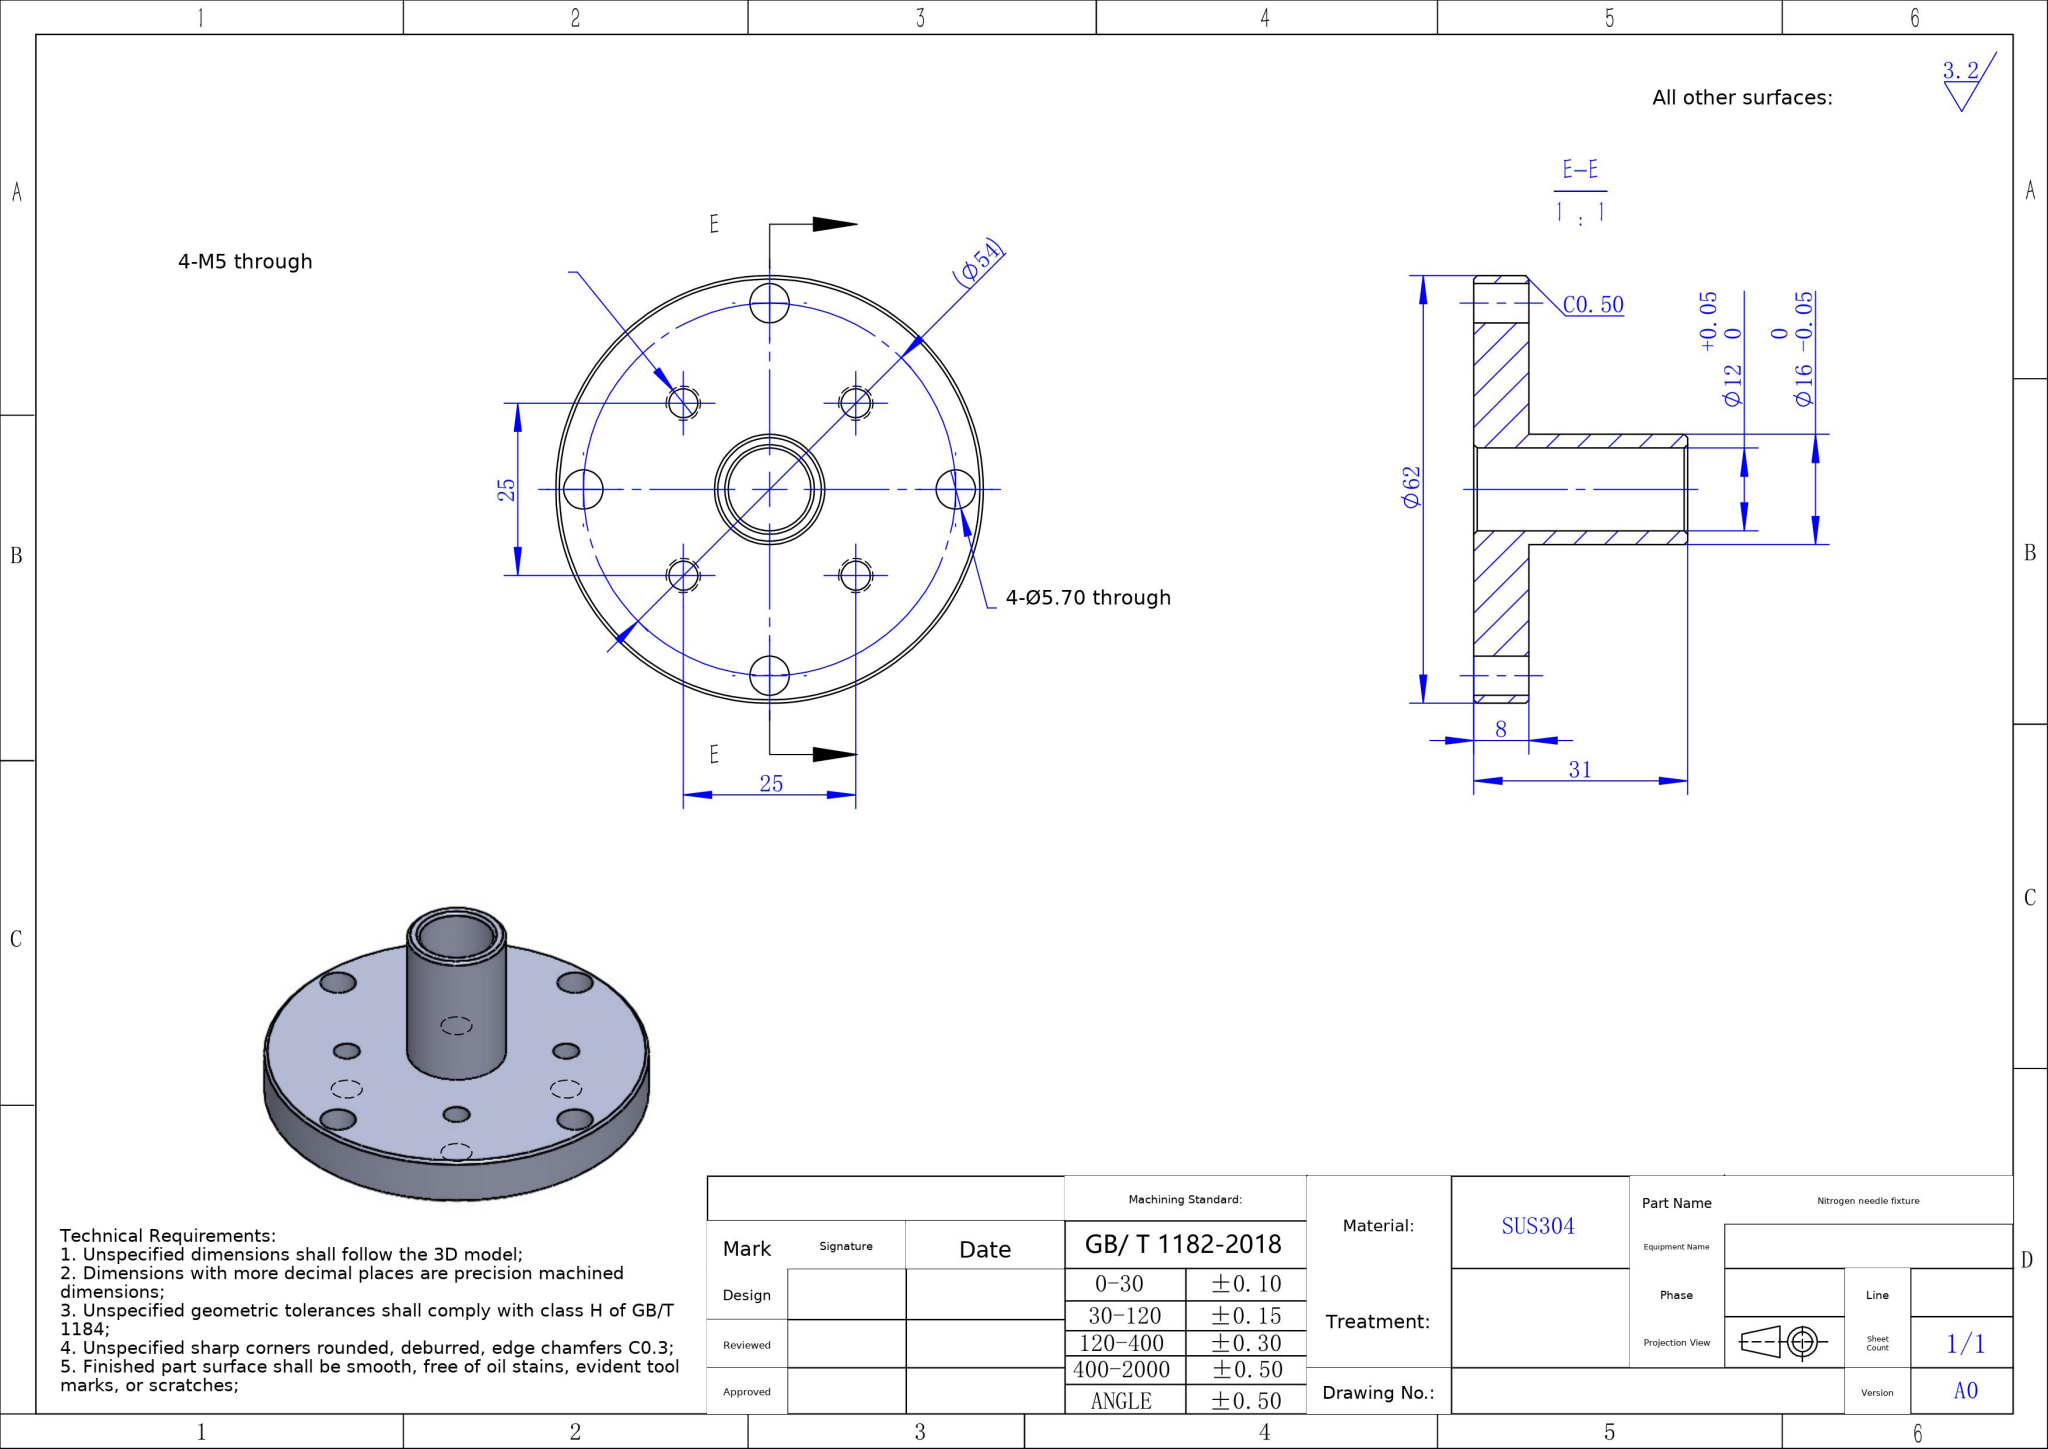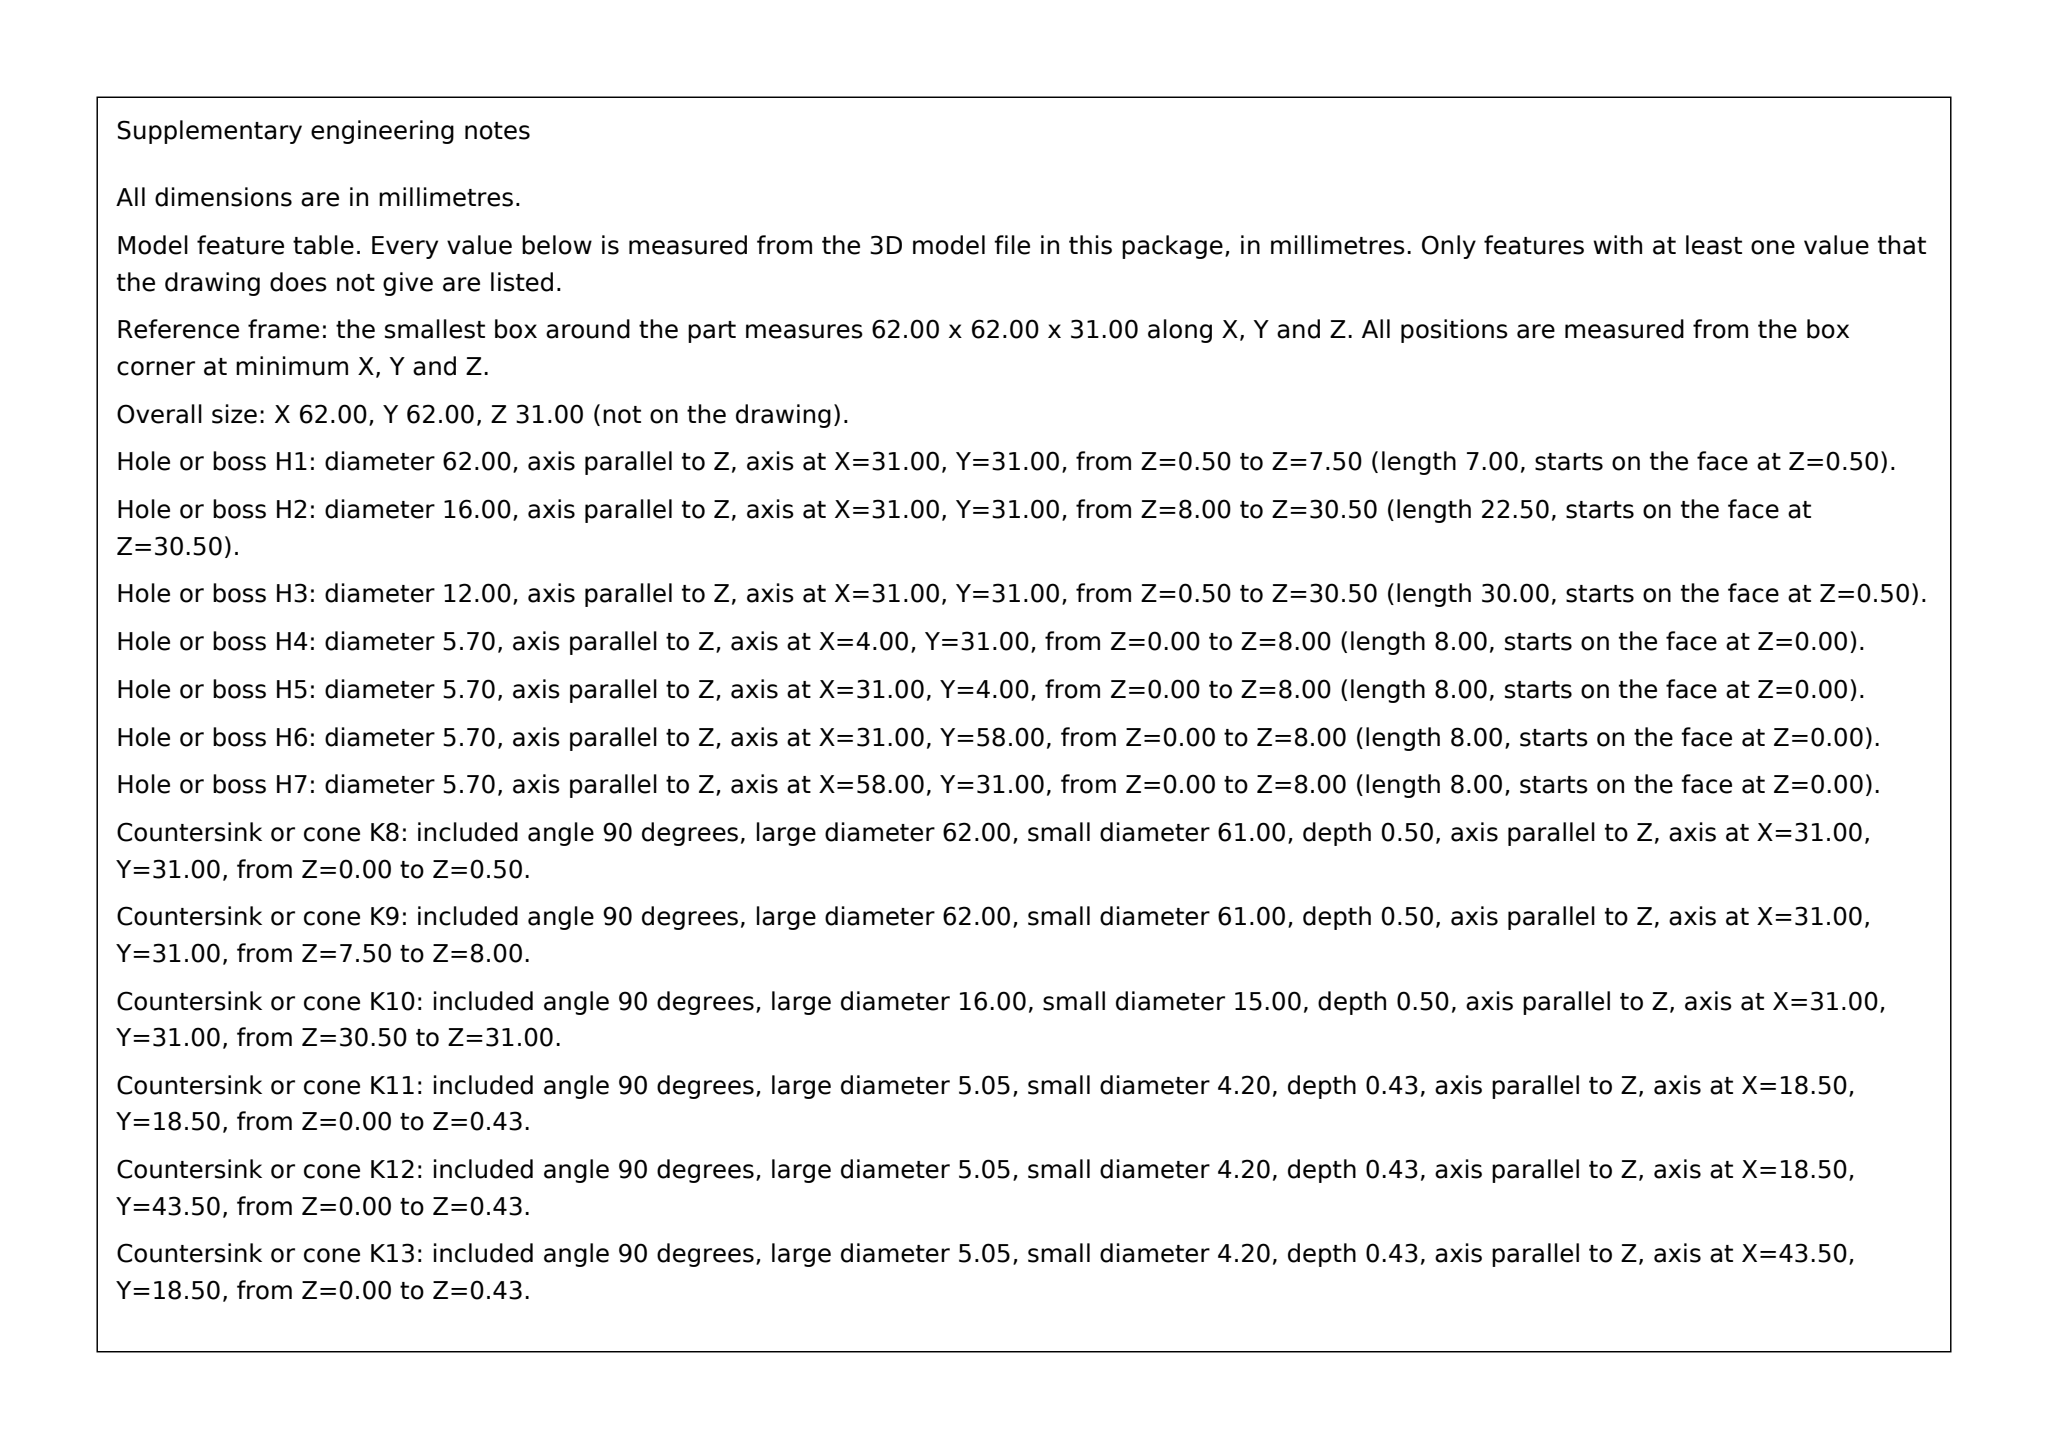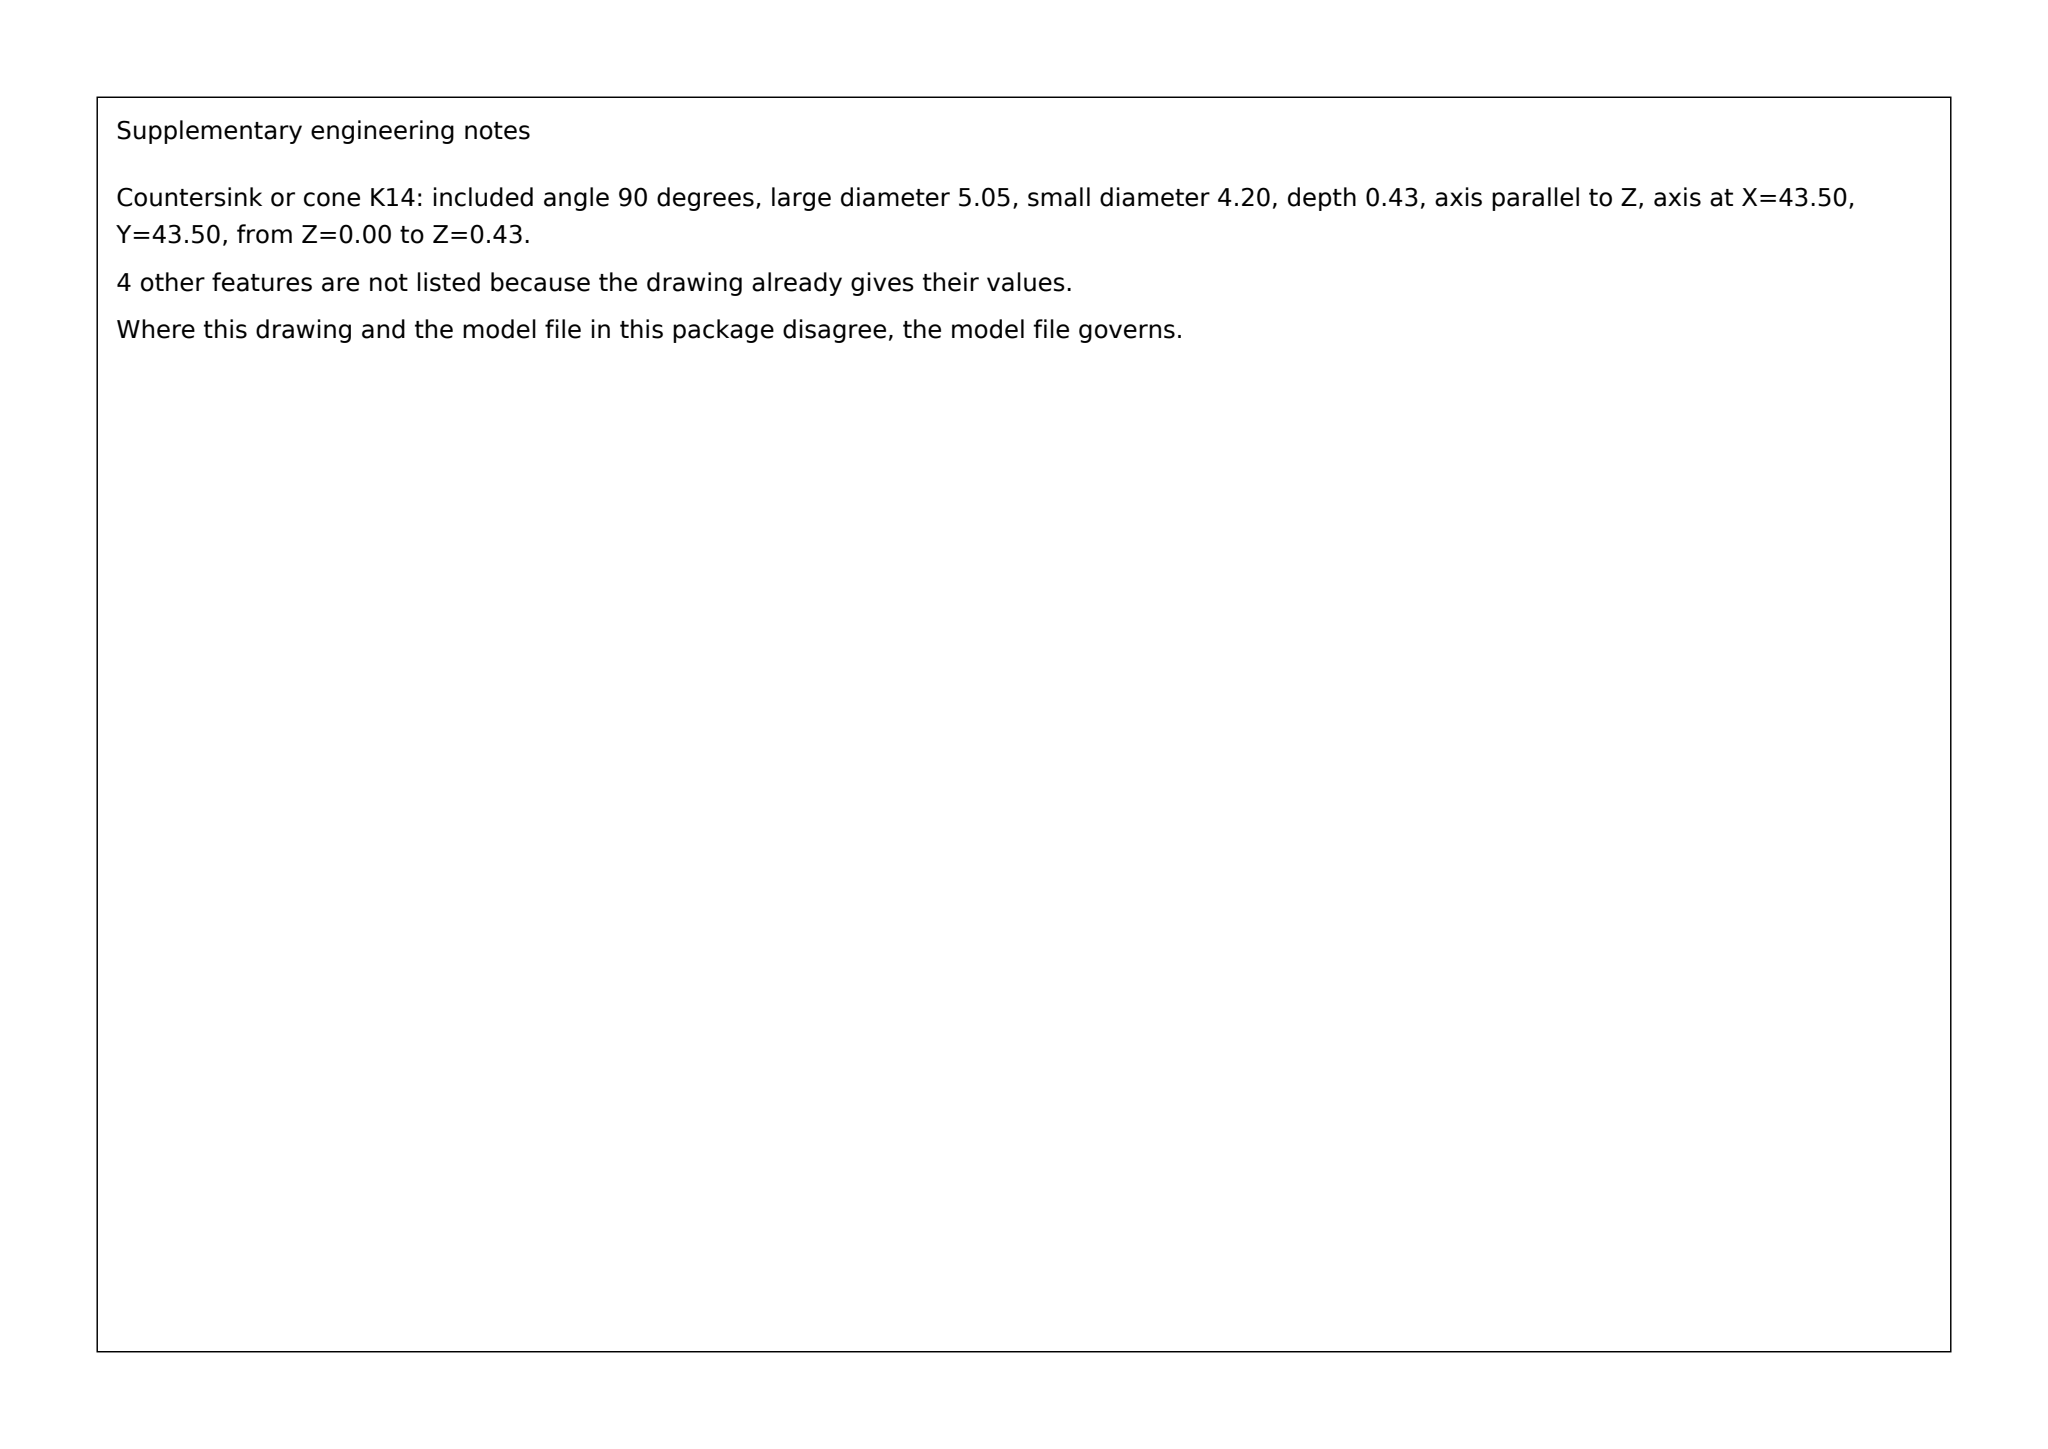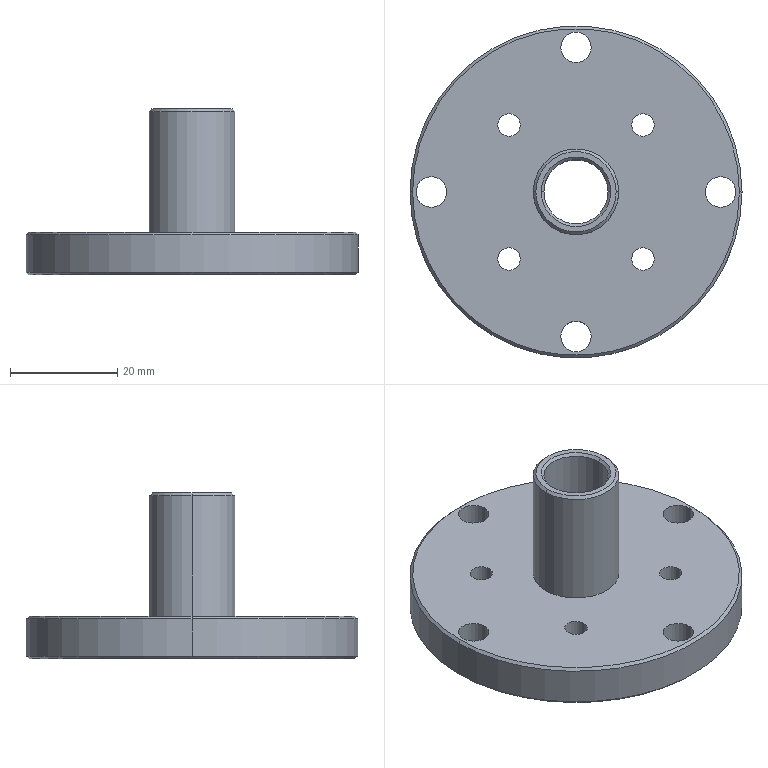Part | SolidWorks | mm | material SUS304 | 1 solid | 43 faces | box 62 x 62 x 31 mm | volume 23942 mm3 | cylinder 22 | cone 18 | plane 3 | commonest cylinder face diameters 4.2 x8 5.7 x8 12 x2 16 x2 62 x2
build123d program:
from build123d import *

# Parameters (mm, degrees)
SKETCH1_R                   = 31
BOSS_EXTRUDE1_DEPTH         = 8
SKETCH2_R                   = 8
BOSS_EXTRUDE2_DEPTH         = 23
SKETCH3_R                   = 6
CUT_EXTRUDE1_DEPTH          = 54.694
CHAMFER1_SIZE               = 0.5
CHAMFER2_SIZE               = 0.5
SKETCH4_R                   = 2.85
CUT_EXTRUDE2_DEPTH          = 25
M5_TAPPED_HOLE2_D           = 4.2
M5_TAPPED_HOLE2_DEPTH       = 17
M5_TAPPED_HOLE2_CSINK_D     = 5.05
M5_TAPPED_HOLE2_CSINK_ANGLE = 90
M5_TAPPED_HOLE2_TIP         = 1.262
CHAMFER3_SIZE               = 0.5


with BuildPart() as part:
    # Sketch1 → Boss-Extrude1 (new body)
    with BuildSketch(Plane.XY):
        Circle(SKETCH1_R)
    extrude(amount=BOSS_EXTRUDE1_DEPTH)

    # Sketch2 → Boss-Extrude2 (add)
    with BuildSketch(Plane.XY.offset(8)):
        Circle(SKETCH2_R)
    extrude(amount=BOSS_EXTRUDE2_DEPTH)

    # Sketch3 → Cut-Extrude1 (cut, through all)
    with BuildSketch(Plane.XY.offset(31)):
        Circle(SKETCH3_R)
    extrude(amount=-CUT_EXTRUDE1_DEPTH, mode=Mode.SUBTRACT)

    # Chamfer1
    chamfer1_edges = [part.edges().sort_by_distance(p)[0] for p in [
        (-31, 0, 0),
        (-31, 0, 8),
    ]]
    chamfer(chamfer1_edges, length=CHAMFER1_SIZE)

    # Chamfer2
    chamfer2_edges = [part.edges().sort_by_distance(p)[0] for p in [
        (-6, 0, 31),
        (-8, 0, 31),
    ]]
    chamfer(chamfer2_edges, length=CHAMFER2_SIZE)

    # Sketch4 → Cut-Extrude2 (cut)
    with BuildSketch(Plane.XY.offset(8)):
        with Locations((0, 27)):
            Circle(SKETCH4_R)
        with Locations((27, 0)):
            Circle(SKETCH4_R)
        with Locations((0, -27)):
            Circle(SKETCH4_R)
        with Locations((-27, 0)):
            Circle(SKETCH4_R)
    extrude(amount=-CUT_EXTRUDE2_DEPTH, mode=Mode.SUBTRACT)

    # M5 Tapped Hole2
    with Locations(Plane(origin=(0, 0, 0), x_dir=(-1, 0, 0), z_dir=(0, 0, -1))):
        with Locations((12.5, 12.5), (-12.5, 12.5), (-12.5, -12.5), (12.5, -12.5)):
            CounterSinkHole(M5_TAPPED_HOLE2_D / 2, M5_TAPPED_HOLE2_CSINK_D / 2, depth=M5_TAPPED_HOLE2_DEPTH, counter_sink_angle=M5_TAPPED_HOLE2_CSINK_ANGLE)
            with Locations((0, 0, -(M5_TAPPED_HOLE2_DEPTH + M5_TAPPED_HOLE2_TIP / 2))):  # 118° drill point
                Cone(0, M5_TAPPED_HOLE2_D / 2, M5_TAPPED_HOLE2_TIP, mode=Mode.SUBTRACT)

    # Chamfer3
    chamfer3_edges = [part.edges().sort_by_distance(p)[0] for p in [
        (-6, 0, 0),
    ]]
    chamfer(chamfer3_edges, length=CHAMFER3_SIZE)


solid = part.part